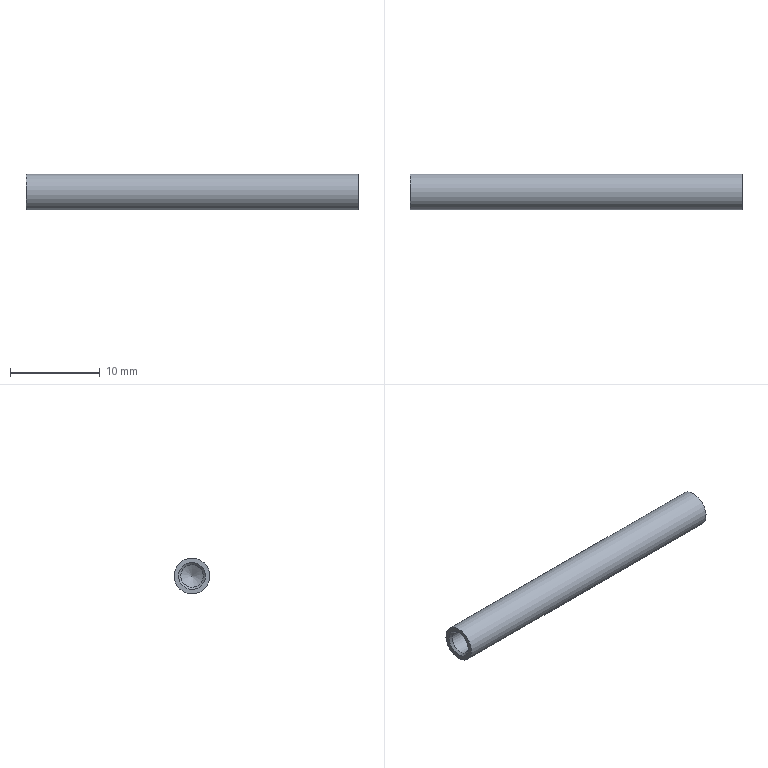Component | NX | DJZ_14_PIN_SHAFT | 1 solid | 9 faces | box 37 x 4 x 4 mm | volume 403 mm3 | cone 4 | cylinder 3 | plane 2 | commonest cylinder face diameters 2.5 x2 4 x1
STEP:
#1=CARTESIAN_POINT('',(0.,0.,0.));
#2=DIRECTION('',(0.,0.,1.));
#3=DIRECTION('',(1.,0.,0.));
#4=AXIS2_PLACEMENT_3D('',#1,#2,#3);
#5=CARTESIAN_POINT('',(29.5,11.348,35.764));
#6=VERTEX_POINT('',#5);
#7=CARTESIAN_POINT('',(29.5,9.5,35.));
#8=DIRECTION('',(1.,0.,0.));
#9=DIRECTION('',(0.,0.9242,0.3818));
#10=AXIS2_PLACEMENT_3D('',#7,#8,#9);
#11=CIRCLE('',#10,2.);
#12=CARTESIAN_POINT('',(29.5,9.5,35.));
#13=DIRECTION('',(-1.,0.,0.));
#14=DIRECTION('',(0.,-0.9242,-0.3818));
#15=AXIS2_PLACEMENT_3D('',#12,#13,#14);
#16=CYLINDRICAL_SURFACE('',#15,2.);
#17=CARTESIAN_POINT('',(9.425,0.));
#18=DIRECTION('',(-1.,0.));
#19=VECTOR('',#18,1.);
#20=LINE('',#17,#19);
#21=(GEOMETRIC_REPRESENTATION_CONTEXT(2)PARAMETRIC_REPRESENTATION_CONTEXT()REPRESENTATION_CONTEXT('',''));
#22=DEFINITIONAL_REPRESENTATION('',(#20),#21);
#23=PCURVE('',#16,#22);
#24=CARTESIAN_POINT('',(29.5,9.5,35.));
#25=DIRECTION('',(1.,0.,0.));
#26=DIRECTION('',(0.,0.9242,0.3818));
#27=AXIS2_PLACEMENT_3D('',#24,#25,#26);
#28=PLANE('',#27);
#29=CARTESIAN_POINT('',(0.,0.));
#30=DIRECTION('',(1.,-0.));
#31=AXIS2_PLACEMENT_2D('',#29,#30);
#32=CIRCLE('',#31,2.);
#33=(GEOMETRIC_REPRESENTATION_CONTEXT(2)PARAMETRIC_REPRESENTATION_CONTEXT()REPRESENTATION_CONTEXT('',''));
#34=DEFINITIONAL_REPRESENTATION('',(#32),#33);
#35=PCURVE('',#28,#34);
#36=SURFACE_CURVE('',#11,(#23,#35),.PCURVE_S1.);
#37=EDGE_CURVE('',#6,#6,#36,.T.);
#38=ORIENTED_EDGE('',*,*,#37,.F.);
#39=CARTESIAN_POINT('',(-7.5,11.348,35.764));
#40=VERTEX_POINT('',#39);
#41=CARTESIAN_POINT('',(29.5,11.348,35.764));
#42=CARTESIAN_POINT('',(-7.5,11.348,35.764));
#43=B_SPLINE_CURVE_WITH_KNOTS('',1,(#41,#42),.UNSPECIFIED.,.F.,.F.,(2,2),(0.,37.),.PIECEWISE_BEZIER_KNOTS.);
#44=CARTESIAN_POINT('',(9.425,0.));
#45=DIRECTION('',(0.,1.));
#46=VECTOR('',#45,1.);
#47=LINE('',#44,#46);
#48=(GEOMETRIC_REPRESENTATION_CONTEXT(2)PARAMETRIC_REPRESENTATION_CONTEXT()REPRESENTATION_CONTEXT('',''));
#49=DEFINITIONAL_REPRESENTATION('',(#47),#48);
#50=PCURVE('',#16,#49);
#51=CARTESIAN_POINT('',(3.142,0.));
#52=DIRECTION('',(0.,1.));
#53=VECTOR('',#52,1.);
#54=LINE('',#51,#53);
#55=(GEOMETRIC_REPRESENTATION_CONTEXT(2)PARAMETRIC_REPRESENTATION_CONTEXT()REPRESENTATION_CONTEXT('',''));
#56=DEFINITIONAL_REPRESENTATION('',(#54),#55);
#57=PCURVE('',#16,#56);
#58=SEAM_CURVE('',#43,(#50,#57),.PCURVE_S1.);
#59=EDGE_CURVE('',#6,#40,#58,.T.);
#60=ORIENTED_EDGE('',*,*,#59,.T.);
#61=CARTESIAN_POINT('',(-7.5,9.5,35.));
#62=DIRECTION('',(1.,0.,0.));
#63=DIRECTION('',(0.,0.9242,0.3818));
#64=AXIS2_PLACEMENT_3D('',#61,#62,#63);
#65=CIRCLE('',#64,2.);
#66=CARTESIAN_POINT('',(9.425,37.));
#67=DIRECTION('',(-1.,0.));
#68=VECTOR('',#67,1.);
#69=LINE('',#66,#68);
#70=(GEOMETRIC_REPRESENTATION_CONTEXT(2)PARAMETRIC_REPRESENTATION_CONTEXT()REPRESENTATION_CONTEXT('',''));
#71=DEFINITIONAL_REPRESENTATION('',(#69),#70);
#72=PCURVE('',#16,#71);
#73=CARTESIAN_POINT('',(-7.5,9.5,35.));
#74=DIRECTION('',(1.,0.,0.));
#75=DIRECTION('',(0.,0.9242,0.3818));
#76=AXIS2_PLACEMENT_3D('',#73,#74,#75);
#77=PLANE('',#76);
#78=CARTESIAN_POINT('',(0.,0.));
#79=DIRECTION('',(1.,-0.));
#80=AXIS2_PLACEMENT_2D('',#78,#79);
#81=CIRCLE('',#80,2.);
#82=(GEOMETRIC_REPRESENTATION_CONTEXT(2)PARAMETRIC_REPRESENTATION_CONTEXT()REPRESENTATION_CONTEXT('',''));
#83=DEFINITIONAL_REPRESENTATION('',(#81),#82);
#84=PCURVE('',#77,#83);
#85=SURFACE_CURVE('',#65,(#72,#84),.PCURVE_S1.);
#86=EDGE_CURVE('',#40,#40,#85,.T.);
#87=ORIENTED_EDGE('',*,*,#86,.T.);
#88=ORIENTED_EDGE('',*,*,#59,.F.);
#89=EDGE_LOOP('',(#38,#60,#87,#88));
#90=FACE_BOUND('',#89,.T.);
#91=ADVANCED_FACE('',(#90),#16,.T.);
#92=CARTESIAN_POINT('',(29.5,10.886,35.573));
#93=VERTEX_POINT('',#92);
#94=CARTESIAN_POINT('',(29.5,9.5,35.));
#95=DIRECTION('',(-1.,0.,0.));
#96=DIRECTION('',(0.,0.9242,0.3818));
#97=AXIS2_PLACEMENT_3D('',#94,#95,#96);
#98=CIRCLE('',#97,1.5);
#99=CARTESIAN_POINT('',(1.5,-0.));
#100=CARTESIAN_POINT('',(1.5,-2.598));
#101=CARTESIAN_POINT('',(-0.75,-1.299));
#102=CARTESIAN_POINT('',(-3.,0.));
#103=CARTESIAN_POINT('',(-0.75,1.299));
#104=CARTESIAN_POINT('',(1.5,2.598));
#105=CARTESIAN_POINT('',(1.5,-0.));
#106=(BOUNDED_CURVE()B_SPLINE_CURVE(2,(#99,#100,#101,#102,#103,#104,#105),.UNSPECIFIED.,.T.,.F.)B_SPLINE_CURVE_WITH_KNOTS((1,2,2,2,2,1),(-2.094,0.,2.094,4.189,6.283,8.378),.UNSPECIFIED.)CURVE()GEOMETRIC_REPRESENTATION_ITEM()RATIONAL_B_SPLINE_CURVE((1.,0.5,1.,0.5,1.,0.5,1.))REPRESENTATION_ITEM(''));
#107=(GEOMETRIC_REPRESENTATION_CONTEXT(2)PARAMETRIC_REPRESENTATION_CONTEXT()REPRESENTATION_CONTEXT('',''));
#108=DEFINITIONAL_REPRESENTATION('',(#106),#107);
#109=PCURVE('',#28,#108);
#110=CARTESIAN_POINT('',(29.5,9.5,35.));
#111=DIRECTION('',(1.,0.,0.));
#112=DIRECTION('',(0.,0.9242,0.3818));
#113=AXIS2_PLACEMENT_3D('',#110,#111,#112);
#114=CONICAL_SURFACE('',#113,1.5,0.7854);
#115=CARTESIAN_POINT('',(6.283,0.));
#116=DIRECTION('',(-1.,0.));
#117=VECTOR('',#116,1.);
#118=LINE('',#115,#117);
#119=(GEOMETRIC_REPRESENTATION_CONTEXT(2)PARAMETRIC_REPRESENTATION_CONTEXT()REPRESENTATION_CONTEXT('',''));
#120=DEFINITIONAL_REPRESENTATION('',(#118),#119);
#121=PCURVE('',#114,#120);
#122=SURFACE_CURVE('',#98,(#109,#121),.PCURVE_S1.);
#123=EDGE_CURVE('',#93,#93,#122,.T.);
#124=ORIENTED_EDGE('',*,*,#123,.T.);
#125=EDGE_LOOP('',(#124));
#126=FACE_BOUND('',#125,.T.);
#127=ORIENTED_EDGE('',*,*,#37,.T.);
#128=EDGE_LOOP('',(#127));
#129=FACE_BOUND('',#128,.T.);
#130=ADVANCED_FACE('',(#126,#129),#28,.T.);
#131=CARTESIAN_POINT('',(-7.5,10.886,35.573));
#132=VERTEX_POINT('',#131);
#133=CARTESIAN_POINT('',(-7.5,9.5,35.));
#134=DIRECTION('',(1.,0.,0.));
#135=DIRECTION('',(0.,0.9242,0.3818));
#136=AXIS2_PLACEMENT_3D('',#133,#134,#135);
#137=CIRCLE('',#136,1.5);
#138=CARTESIAN_POINT('',(0.,0.));
#139=DIRECTION('',(1.,-0.));
#140=AXIS2_PLACEMENT_2D('',#138,#139);
#141=CIRCLE('',#140,1.5);
#142=(GEOMETRIC_REPRESENTATION_CONTEXT(2)PARAMETRIC_REPRESENTATION_CONTEXT()REPRESENTATION_CONTEXT('',''));
#143=DEFINITIONAL_REPRESENTATION('',(#141),#142);
#144=PCURVE('',#77,#143);
#145=CARTESIAN_POINT('',(-7.5,9.5,35.));
#146=DIRECTION('',(-1.,0.,0.));
#147=DIRECTION('',(0.,-0.9242,-0.3818));
#148=AXIS2_PLACEMENT_3D('',#145,#146,#147);
#149=CONICAL_SURFACE('',#148,1.5,0.7854);
#150=CARTESIAN_POINT('',(9.425,0.));
#151=DIRECTION('',(-1.,0.));
#152=VECTOR('',#151,1.);
#153=LINE('',#150,#152);
#154=(GEOMETRIC_REPRESENTATION_CONTEXT(2)PARAMETRIC_REPRESENTATION_CONTEXT()REPRESENTATION_CONTEXT('',''));
#155=DEFINITIONAL_REPRESENTATION('',(#153),#154);
#156=PCURVE('',#149,#155);
#157=SURFACE_CURVE('',#137,(#144,#156),.PCURVE_S1.);
#158=EDGE_CURVE('',#132,#132,#157,.T.);
#159=ORIENTED_EDGE('',*,*,#158,.T.);
#160=EDGE_LOOP('',(#159));
#161=FACE_BOUND('',#160,.T.);
#162=ORIENTED_EDGE('',*,*,#86,.F.);
#163=EDGE_LOOP('',(#162));
#164=FACE_BOUND('',#163,.T.);
#165=ADVANCED_FACE('',(#161,#164),#77,.F.);
#166=CARTESIAN_POINT('',(23.5,10.655,35.477));
#167=VERTEX_POINT('',#166);
#168=CARTESIAN_POINT('',(23.5,8.345,34.523));
#169=VERTEX_POINT('',#168);
#170=CARTESIAN_POINT('',(23.5,9.5,35.));
#171=DIRECTION('',(1.,0.,0.));
#172=DIRECTION('',(0.,-0.9242,-0.3818));
#173=AXIS2_PLACEMENT_3D('',#170,#171,#172);
#174=CIRCLE('',#173,1.25);
#175=CARTESIAN_POINT('',(23.5,9.5,35.));
#176=DIRECTION('',(1.,0.,0.));
#177=DIRECTION('',(0.,0.9242,0.3818));
#178=AXIS2_PLACEMENT_3D('',#175,#176,#177);
#179=CONICAL_SURFACE('',#178,1.25,1.03);
#180=CARTESIAN_POINT('',(-3.142,0.));
#181=DIRECTION('',(1.,0.));
#182=VECTOR('',#181,1.);
#183=LINE('',#180,#182);
#184=(GEOMETRIC_REPRESENTATION_CONTEXT(2)PARAMETRIC_REPRESENTATION_CONTEXT()REPRESENTATION_CONTEXT('',''));
#185=DEFINITIONAL_REPRESENTATION('',(#183),#184);
#186=PCURVE('',#179,#185);
#187=CARTESIAN_POINT('',(29.5,9.5,35.));
#188=DIRECTION('',(-1.,0.,0.));
#189=DIRECTION('',(0.,-0.9242,-0.3818));
#190=AXIS2_PLACEMENT_3D('',#187,#188,#189);
#191=CYLINDRICAL_SURFACE('',#190,1.25);
#192=CARTESIAN_POINT('',(12.566,6.));
#193=DIRECTION('',(-1.,0.));
#194=VECTOR('',#193,1.);
#195=LINE('',#192,#194);
#196=(GEOMETRIC_REPRESENTATION_CONTEXT(2)PARAMETRIC_REPRESENTATION_CONTEXT()REPRESENTATION_CONTEXT('',''));
#197=DEFINITIONAL_REPRESENTATION('',(#195),#196);
#198=PCURVE('',#191,#197);
#199=SURFACE_CURVE('',#174,(#186,#198),.PCURVE_S1.);
#200=EDGE_CURVE('',#167,#169,#199,.T.);
#201=ORIENTED_EDGE('',*,*,#200,.F.);
#202=CARTESIAN_POINT('',(22.749,9.5,35.));
#203=VERTEX_POINT('',#202);
#204=CARTESIAN_POINT('',(22.749,9.5,35.));
#205=CARTESIAN_POINT('',(23.5,10.655,35.477));
#206=B_SPLINE_CURVE_WITH_KNOTS('',1,(#204,#205),.UNSPECIFIED.,.F.,.F.,(2,2),(-1.458,0.),.PIECEWISE_BEZIER_KNOTS.);
#207=CARTESIAN_POINT('',(0.,0.));
#208=DIRECTION('',(0.,1.));
#209=VECTOR('',#208,1.);
#210=LINE('',#207,#209);
#211=(GEOMETRIC_REPRESENTATION_CONTEXT(2)PARAMETRIC_REPRESENTATION_CONTEXT()REPRESENTATION_CONTEXT('',''));
#212=DEFINITIONAL_REPRESENTATION('',(#210),#211);
#213=PCURVE('',#179,#212);
#214=CARTESIAN_POINT('',(6.283,0.));
#215=DIRECTION('',(0.,1.));
#216=VECTOR('',#215,1.);
#217=LINE('',#214,#216);
#218=(GEOMETRIC_REPRESENTATION_CONTEXT(2)PARAMETRIC_REPRESENTATION_CONTEXT()REPRESENTATION_CONTEXT('',''));
#219=DEFINITIONAL_REPRESENTATION('',(#217),#218);
#220=PCURVE('',#179,#219);
#221=SEAM_CURVE('',#206,(#213,#220),.PCURVE_S1.);
#222=EDGE_CURVE('',#203,#167,#221,.T.);
#223=ORIENTED_EDGE('',*,*,#222,.F.);
#224=ORIENTED_EDGE('',*,*,#222,.T.);
#225=CARTESIAN_POINT('',(23.5,9.5,35.));
#226=DIRECTION('',(1.,0.,0.));
#227=DIRECTION('',(0.,-0.9242,-0.3818));
#228=AXIS2_PLACEMENT_3D('',#225,#226,#227);
#229=CIRCLE('',#228,1.25);
#230=CARTESIAN_POINT('',(3.142,0.));
#231=DIRECTION('',(1.,0.));
#232=VECTOR('',#231,1.);
#233=LINE('',#230,#232);
#234=(GEOMETRIC_REPRESENTATION_CONTEXT(2)PARAMETRIC_REPRESENTATION_CONTEXT()REPRESENTATION_CONTEXT('',''));
#235=DEFINITIONAL_REPRESENTATION('',(#233),#234);
#236=PCURVE('',#179,#235);
#237=CARTESIAN_POINT('',(6.283,6.));
#238=DIRECTION('',(-1.,0.));
#239=VECTOR('',#238,1.);
#240=LINE('',#237,#239);
#241=(GEOMETRIC_REPRESENTATION_CONTEXT(2)PARAMETRIC_REPRESENTATION_CONTEXT()REPRESENTATION_CONTEXT('',''));
#242=DEFINITIONAL_REPRESENTATION('',(#240),#241);
#243=PCURVE('',#191,#242);
#244=SURFACE_CURVE('',#229,(#236,#243),.PCURVE_S1.);
#245=EDGE_CURVE('',#169,#167,#244,.T.);
#246=ORIENTED_EDGE('',*,*,#245,.F.);
#247=EDGE_LOOP('',(#201,#223,#224,#246));
#248=FACE_BOUND('',#247,.F.);
#249=ADVANCED_FACE('',(#248),#179,.F.);
#250=CARTESIAN_POINT('',(29.25,10.655,35.477));
#251=VERTEX_POINT('',#250);
#252=CARTESIAN_POINT('',(29.25,9.5,35.));
#253=DIRECTION('',(1.,0.,0.));
#254=DIRECTION('',(0.,0.9242,0.3818));
#255=AXIS2_PLACEMENT_3D('',#252,#253,#254);
#256=CIRCLE('',#255,1.25);
#257=CARTESIAN_POINT('',(9.425,0.25));
#258=DIRECTION('',(-1.,0.));
#259=VECTOR('',#258,1.);
#260=LINE('',#257,#259);
#261=(GEOMETRIC_REPRESENTATION_CONTEXT(2)PARAMETRIC_REPRESENTATION_CONTEXT()REPRESENTATION_CONTEXT('',''));
#262=DEFINITIONAL_REPRESENTATION('',(#260),#261);
#263=PCURVE('',#191,#262);
#264=CARTESIAN_POINT('',(0.,-0.25));
#265=DIRECTION('',(1.,0.));
#266=VECTOR('',#265,1.);
#267=LINE('',#264,#266);
#268=(GEOMETRIC_REPRESENTATION_CONTEXT(2)PARAMETRIC_REPRESENTATION_CONTEXT()REPRESENTATION_CONTEXT('',''));
#269=DEFINITIONAL_REPRESENTATION('',(#267),#268);
#270=PCURVE('',#114,#269);
#271=SURFACE_CURVE('',#256,(#263,#270),.PCURVE_S1.);
#272=EDGE_CURVE('',#251,#251,#271,.T.);
#273=ORIENTED_EDGE('',*,*,#272,.F.);
#274=CARTESIAN_POINT('',(29.25,10.655,35.477));
#275=CARTESIAN_POINT('',(23.5,10.655,35.477));
#276=B_SPLINE_CURVE_WITH_KNOTS('',1,(#274,#275),.UNSPECIFIED.,.F.,.F.,(2,2),(0.25,6.),.PIECEWISE_BEZIER_KNOTS.);
#277=CARTESIAN_POINT('',(9.425,0.));
#278=DIRECTION('',(0.,1.));
#279=VECTOR('',#278,1.);
#280=LINE('',#277,#279);
#281=(GEOMETRIC_REPRESENTATION_CONTEXT(2)PARAMETRIC_REPRESENTATION_CONTEXT()REPRESENTATION_CONTEXT('',''));
#282=DEFINITIONAL_REPRESENTATION('',(#280),#281);
#283=PCURVE('',#191,#282);
#284=CARTESIAN_POINT('',(3.142,0.));
#285=DIRECTION('',(0.,1.));
#286=VECTOR('',#285,1.);
#287=LINE('',#284,#286);
#288=(GEOMETRIC_REPRESENTATION_CONTEXT(2)PARAMETRIC_REPRESENTATION_CONTEXT()REPRESENTATION_CONTEXT('',''));
#289=DEFINITIONAL_REPRESENTATION('',(#287),#288);
#290=PCURVE('',#191,#289);
#291=SEAM_CURVE('',#276,(#283,#290),.PCURVE_S1.);
#292=EDGE_CURVE('',#251,#167,#291,.T.);
#293=ORIENTED_EDGE('',*,*,#292,.T.);
#294=ORIENTED_EDGE('',*,*,#200,.T.);
#295=ORIENTED_EDGE('',*,*,#245,.T.);
#296=ORIENTED_EDGE('',*,*,#292,.F.);
#297=EDGE_LOOP('',(#273,#293,#294,#295,#296));
#298=FACE_BOUND('',#297,.F.);
#299=ADVANCED_FACE('',(#298),#191,.F.);
#300=ORIENTED_EDGE('',*,*,#272,.T.);
#301=CARTESIAN_POINT('',(29.25,10.655,35.477));
#302=CARTESIAN_POINT('',(29.5,10.886,35.573));
#303=B_SPLINE_CURVE_WITH_KNOTS('',1,(#301,#302),.UNSPECIFIED.,.F.,.F.,(2,2),(-0.3536,0.),.PIECEWISE_BEZIER_KNOTS.);
#304=CARTESIAN_POINT('',(6.283,0.));
#305=DIRECTION('',(0.,1.));
#306=VECTOR('',#305,1.);
#307=LINE('',#304,#306);
#308=(GEOMETRIC_REPRESENTATION_CONTEXT(2)PARAMETRIC_REPRESENTATION_CONTEXT()REPRESENTATION_CONTEXT('',''));
#309=DEFINITIONAL_REPRESENTATION('',(#307),#308);
#310=PCURVE('',#114,#309);
#311=CARTESIAN_POINT('',(0.,0.));
#312=DIRECTION('',(0.,1.));
#313=VECTOR('',#312,1.);
#314=LINE('',#311,#313);
#315=(GEOMETRIC_REPRESENTATION_CONTEXT(2)PARAMETRIC_REPRESENTATION_CONTEXT()REPRESENTATION_CONTEXT('',''));
#316=DEFINITIONAL_REPRESENTATION('',(#314),#315);
#317=PCURVE('',#114,#316);
#318=SEAM_CURVE('',#303,(#310,#317),.PCURVE_S1.);
#319=EDGE_CURVE('',#251,#93,#318,.T.);
#320=ORIENTED_EDGE('',*,*,#319,.T.);
#321=ORIENTED_EDGE('',*,*,#123,.T.);
#322=ORIENTED_EDGE('',*,*,#319,.F.);
#323=EDGE_LOOP('',(#300,#320,#321,#322));
#324=FACE_BOUND('',#323,.F.);
#325=ADVANCED_FACE('',(#324),#114,.F.);
#326=CARTESIAN_POINT('',(-1.5,8.345,34.523));
#327=VERTEX_POINT('',#326);
#328=CARTESIAN_POINT('',(-1.5,10.655,35.477));
#329=VERTEX_POINT('',#328);
#330=CARTESIAN_POINT('',(-1.5,9.5,35.));
#331=DIRECTION('',(-1.,0.,0.));
#332=DIRECTION('',(0.,0.9242,0.3818));
#333=AXIS2_PLACEMENT_3D('',#330,#331,#332);
#334=CIRCLE('',#333,1.25);
#335=CARTESIAN_POINT('',(-1.5,9.5,35.));
#336=DIRECTION('',(-1.,0.,0.));
#337=DIRECTION('',(0.,-0.9242,-0.3818));
#338=AXIS2_PLACEMENT_3D('',#335,#336,#337);
#339=CONICAL_SURFACE('',#338,1.25,1.03);
#340=CARTESIAN_POINT('',(-3.142,0.));
#341=DIRECTION('',(1.,0.));
#342=VECTOR('',#341,1.);
#343=LINE('',#340,#342);
#344=(GEOMETRIC_REPRESENTATION_CONTEXT(2)PARAMETRIC_REPRESENTATION_CONTEXT()REPRESENTATION_CONTEXT('',''));
#345=DEFINITIONAL_REPRESENTATION('',(#343),#344);
#346=PCURVE('',#339,#345);
#347=CARTESIAN_POINT('',(-7.5,9.5,35.));
#348=DIRECTION('',(1.,0.,0.));
#349=DIRECTION('',(0.,0.9242,0.3818));
#350=AXIS2_PLACEMENT_3D('',#347,#348,#349);
#351=CYLINDRICAL_SURFACE('',#350,1.25);
#352=CARTESIAN_POINT('',(6.283,6.));
#353=DIRECTION('',(-1.,0.));
#354=VECTOR('',#353,1.);
#355=LINE('',#352,#354);
#356=(GEOMETRIC_REPRESENTATION_CONTEXT(2)PARAMETRIC_REPRESENTATION_CONTEXT()REPRESENTATION_CONTEXT('',''));
#357=DEFINITIONAL_REPRESENTATION('',(#355),#356);
#358=PCURVE('',#351,#357);
#359=SURFACE_CURVE('',#334,(#346,#358),.PCURVE_S1.);
#360=EDGE_CURVE('',#327,#329,#359,.T.);
#361=ORIENTED_EDGE('',*,*,#360,.F.);
#362=CARTESIAN_POINT('',(-0.7489,9.5,35.));
#363=VERTEX_POINT('',#362);
#364=CARTESIAN_POINT('',(-0.7489,9.5,35.));
#365=CARTESIAN_POINT('',(-1.5,8.345,34.523));
#366=B_SPLINE_CURVE_WITH_KNOTS('',1,(#364,#365),.UNSPECIFIED.,.F.,.F.,(2,2),(-1.458,0.),.PIECEWISE_BEZIER_KNOTS.);
#367=CARTESIAN_POINT('',(0.,0.));
#368=DIRECTION('',(0.,1.));
#369=VECTOR('',#368,1.);
#370=LINE('',#367,#369);
#371=(GEOMETRIC_REPRESENTATION_CONTEXT(2)PARAMETRIC_REPRESENTATION_CONTEXT()REPRESENTATION_CONTEXT('',''));
#372=DEFINITIONAL_REPRESENTATION('',(#370),#371);
#373=PCURVE('',#339,#372);
#374=CARTESIAN_POINT('',(6.283,0.));
#375=DIRECTION('',(0.,1.));
#376=VECTOR('',#375,1.);
#377=LINE('',#374,#376);
#378=(GEOMETRIC_REPRESENTATION_CONTEXT(2)PARAMETRIC_REPRESENTATION_CONTEXT()REPRESENTATION_CONTEXT('',''));
#379=DEFINITIONAL_REPRESENTATION('',(#377),#378);
#380=PCURVE('',#339,#379);
#381=SEAM_CURVE('',#366,(#373,#380),.PCURVE_S1.);
#382=EDGE_CURVE('',#363,#327,#381,.T.);
#383=ORIENTED_EDGE('',*,*,#382,.F.);
#384=ORIENTED_EDGE('',*,*,#382,.T.);
#385=CARTESIAN_POINT('',(-1.5,9.5,35.));
#386=DIRECTION('',(-1.,0.,0.));
#387=DIRECTION('',(0.,0.9242,0.3818));
#388=AXIS2_PLACEMENT_3D('',#385,#386,#387);
#389=CIRCLE('',#388,1.25);
#390=CARTESIAN_POINT('',(3.142,0.));
#391=DIRECTION('',(1.,0.));
#392=VECTOR('',#391,1.);
#393=LINE('',#390,#392);
#394=(GEOMETRIC_REPRESENTATION_CONTEXT(2)PARAMETRIC_REPRESENTATION_CONTEXT()REPRESENTATION_CONTEXT('',''));
#395=DEFINITIONAL_REPRESENTATION('',(#393),#394);
#396=PCURVE('',#339,#395);
#397=CARTESIAN_POINT('',(6.283,6.));
#398=DIRECTION('',(-1.,0.));
#399=VECTOR('',#398,1.);
#400=LINE('',#397,#399);
#401=(GEOMETRIC_REPRESENTATION_CONTEXT(2)PARAMETRIC_REPRESENTATION_CONTEXT()REPRESENTATION_CONTEXT('',''));
#402=DEFINITIONAL_REPRESENTATION('',(#400),#401);
#403=PCURVE('',#351,#402);
#404=SURFACE_CURVE('',#389,(#396,#403),.PCURVE_S1.);
#405=EDGE_CURVE('',#329,#327,#404,.T.);
#406=ORIENTED_EDGE('',*,*,#405,.F.);
#407=EDGE_LOOP('',(#361,#383,#384,#406));
#408=FACE_BOUND('',#407,.F.);
#409=ADVANCED_FACE('',(#408),#339,.F.);
#410=CARTESIAN_POINT('',(-7.25,10.655,35.477));
#411=VERTEX_POINT('',#410);
#412=CARTESIAN_POINT('',(-7.25,9.5,35.));
#413=DIRECTION('',(-1.,0.,0.));
#414=DIRECTION('',(0.,0.9242,0.3818));
#415=AXIS2_PLACEMENT_3D('',#412,#413,#414);
#416=CIRCLE('',#415,1.25);
#417=CARTESIAN_POINT('',(6.283,0.25));
#418=DIRECTION('',(-1.,0.));
#419=VECTOR('',#418,1.);
#420=LINE('',#417,#419);
#421=(GEOMETRIC_REPRESENTATION_CONTEXT(2)PARAMETRIC_REPRESENTATION_CONTEXT()REPRESENTATION_CONTEXT('',''));
#422=DEFINITIONAL_REPRESENTATION('',(#420),#421);
#423=PCURVE('',#351,#422);
#424=CARTESIAN_POINT('',(3.142,-0.25));
#425=DIRECTION('',(1.,0.));
#426=VECTOR('',#425,1.);
#427=LINE('',#424,#426);
#428=(GEOMETRIC_REPRESENTATION_CONTEXT(2)PARAMETRIC_REPRESENTATION_CONTEXT()REPRESENTATION_CONTEXT('',''));
#429=DEFINITIONAL_REPRESENTATION('',(#427),#428);
#430=PCURVE('',#149,#429);
#431=SURFACE_CURVE('',#416,(#423,#430),.PCURVE_S1.);
#432=EDGE_CURVE('',#411,#411,#431,.T.);
#433=ORIENTED_EDGE('',*,*,#432,.F.);
#434=CARTESIAN_POINT('',(-7.25,10.655,35.477));
#435=CARTESIAN_POINT('',(-1.5,10.655,35.477));
#436=B_SPLINE_CURVE_WITH_KNOTS('',1,(#434,#435),.UNSPECIFIED.,.F.,.F.,(2,2),(0.25,6.),.PIECEWISE_BEZIER_KNOTS.);
#437=CARTESIAN_POINT('',(6.283,0.));
#438=DIRECTION('',(0.,1.));
#439=VECTOR('',#438,1.);
#440=LINE('',#437,#439);
#441=(GEOMETRIC_REPRESENTATION_CONTEXT(2)PARAMETRIC_REPRESENTATION_CONTEXT()REPRESENTATION_CONTEXT('',''));
#442=DEFINITIONAL_REPRESENTATION('',(#440),#441);
#443=PCURVE('',#351,#442);
#444=CARTESIAN_POINT('',(0.,0.));
#445=DIRECTION('',(0.,1.));
#446=VECTOR('',#445,1.);
#447=LINE('',#444,#446);
#448=(GEOMETRIC_REPRESENTATION_CONTEXT(2)PARAMETRIC_REPRESENTATION_CONTEXT()REPRESENTATION_CONTEXT('',''));
#449=DEFINITIONAL_REPRESENTATION('',(#447),#448);
#450=PCURVE('',#351,#449);
#451=SEAM_CURVE('',#436,(#443,#450),.PCURVE_S1.);
#452=EDGE_CURVE('',#411,#329,#451,.T.);
#453=ORIENTED_EDGE('',*,*,#452,.T.);
#454=ORIENTED_EDGE('',*,*,#405,.T.);
#455=ORIENTED_EDGE('',*,*,#360,.T.);
#456=ORIENTED_EDGE('',*,*,#452,.F.);
#457=EDGE_LOOP('',(#433,#453,#454,#455,#456));
#458=FACE_BOUND('',#457,.F.);
#459=ADVANCED_FACE('',(#458),#351,.F.);
#460=ORIENTED_EDGE('',*,*,#432,.T.);
#461=CARTESIAN_POINT('',(-7.25,10.655,35.477));
#462=CARTESIAN_POINT('',(-7.5,10.886,35.573));
#463=B_SPLINE_CURVE_WITH_KNOTS('',1,(#461,#462),.UNSPECIFIED.,.F.,.F.,(2,2),(-0.3536,0.),.PIECEWISE_BEZIER_KNOTS.);
#464=CARTESIAN_POINT('',(9.425,0.));
#465=DIRECTION('',(0.,1.));
#466=VECTOR('',#465,1.);
#467=LINE('',#464,#466);
#468=(GEOMETRIC_REPRESENTATION_CONTEXT(2)PARAMETRIC_REPRESENTATION_CONTEXT()REPRESENTATION_CONTEXT('',''));
#469=DEFINITIONAL_REPRESENTATION('',(#467),#468);
#470=PCURVE('',#149,#469);
#471=CARTESIAN_POINT('',(3.142,0.));
#472=DIRECTION('',(0.,1.));
#473=VECTOR('',#472,1.);
#474=LINE('',#471,#473);
#475=(GEOMETRIC_REPRESENTATION_CONTEXT(2)PARAMETRIC_REPRESENTATION_CONTEXT()REPRESENTATION_CONTEXT('',''));
#476=DEFINITIONAL_REPRESENTATION('',(#474),#475);
#477=PCURVE('',#149,#476);
#478=SEAM_CURVE('',#463,(#470,#477),.PCURVE_S1.);
#479=EDGE_CURVE('',#411,#132,#478,.T.);
#480=ORIENTED_EDGE('',*,*,#479,.T.);
#481=ORIENTED_EDGE('',*,*,#158,.T.);
#482=ORIENTED_EDGE('',*,*,#479,.F.);
#483=EDGE_LOOP('',(#460,#480,#481,#482));
#484=FACE_BOUND('',#483,.F.);
#485=ADVANCED_FACE('',(#484),#149,.F.);
#486=CLOSED_SHELL('',(#91,#130,#165,#249,#299,#325,#409,#459,#485));
#487=MANIFOLD_SOLID_BREP('',#486);
#488=(LENGTH_UNIT()NAMED_UNIT(*)SI_UNIT(.MILLI.,.METRE.));
#489=UNCERTAINTY_MEASURE_WITH_UNIT(LENGTH_MEASURE(0.00001),#488,'','');
#490=(NAMED_UNIT(*)PLANE_ANGLE_UNIT()SI_UNIT($,.RADIAN.));
#491=(NAMED_UNIT(*)SI_UNIT($,.STERADIAN.)SOLID_ANGLE_UNIT());
#492=(GEOMETRIC_REPRESENTATION_CONTEXT(3)GLOBAL_UNCERTAINTY_ASSIGNED_CONTEXT((#489))GLOBAL_UNIT_ASSIGNED_CONTEXT((#488,#490,#491))REPRESENTATION_CONTEXT('',''));
#493=ADVANCED_BREP_SHAPE_REPRESENTATION('',(#4,#487),#492);